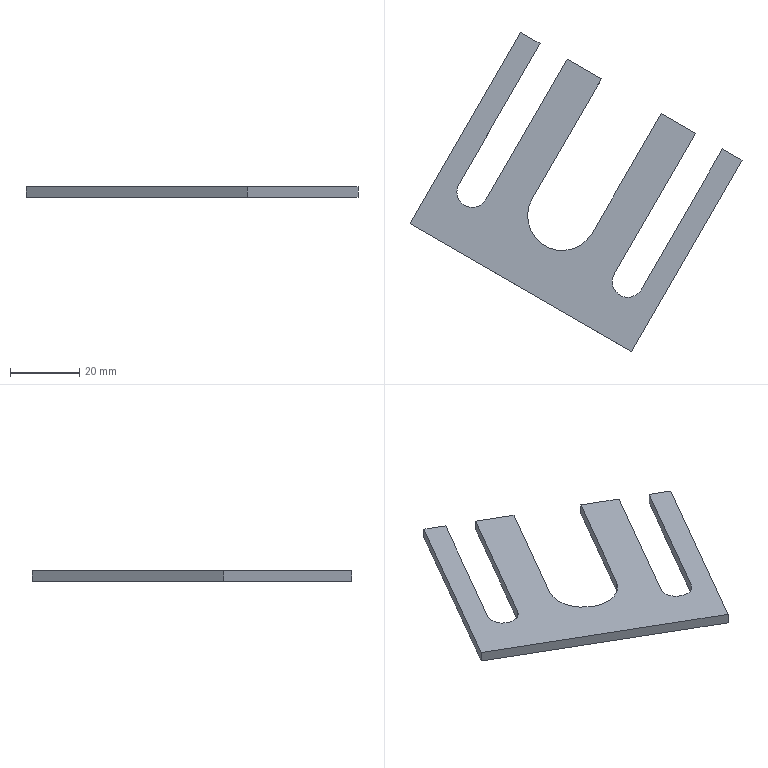Component | SolidWorks | KLHFH018AdjustmentShim-1 | 1 solid | 18 faces | box 96.09 x 92.43 x 3 mm | volume 8608 mm3 | plane 15 | cylinder 3 | commonest cylinder face diameters 9 x2 20 x1 | material AISI 304
build123d program:
from build123d import *

# Parameters (mm, degrees)
SKETCH1_W           = 74
SKETCH1_H           = 64
BOSS_EXTRUDE1_DEPTH = 1.5
SKETCH2_R           = 8
CUT_EXTRUDE1_DEPTH  = 50.01
M8_TAPPED_HOLE1_D   = 6.8
CIRPATTERN1_COUNT   = 6
CUT_EXTRUDE2_DEPTH  = 50.01


with BuildPart() as part:
    # Sketch1 → Boss-Extrude1 (new, symmetric)
    with BuildSketch(Plane.XY):
        Rectangle(SKETCH1_W, SKETCH1_H)
    extrude(amount=BOSS_EXTRUDE1_DEPTH, both=True)

    # Sketch2 → Cut-Extrude1 (cut, through all)
    with BuildSketch(Plane.XY.offset(1.5)):
        Circle(SKETCH2_R)
    extrude(amount=-CUT_EXTRUDE1_DEPTH, mode=Mode.SUBTRACT)

    # M8 Tapped Hole1 (through all)
    with Locations(Plane(origin=(0, 0, -1.5), x_dir=(-1, 0, 0), z_dir=(0, 0, -1))):
        with Locations((-25.981, 15)):
            m8_tapped_hole1 = Hole(M8_TAPPED_HOLE1_D / 2)

    # CirPattern1: M8 Tapped Hole1 ×6 about axis, 2 skipped
    cirpattern1_axis = Axis((0, 0, -1.5), (0, 0, 1))
    add([m8_tapped_hole1.rotate(cirpattern1_axis, i * 360 / CIRPATTERN1_COUNT) for i in range(1, CIRPATTERN1_COUNT) if i not in (1, 4)], mode=Mode.SUBTRACT)

    # Sketch7 → Cut-Extrude2 (cut, through all)
    with BuildSketch(Plane.XY.offset(1.5)):
        with BuildLine():
            Line((-21.481, 15), (-21.481, -32))
            ThreePointArc((-21.481, -32), (-25.981, -36.5), (-30.481, -32))
            Line((-30.481, -32), (-30.481, 15))
            ThreePointArc((-30.481, 15), (-25.981, 19.5), (-21.481, 15))
        make_face()
        with BuildLine():
            Line((30.481, 15), (30.481, -32))
            ThreePointArc((30.481, -32), (25.981, -36.5), (21.481, -32))
            Line((21.481, -32), (21.481, 15))
            ThreePointArc((21.481, 15), (25.981, 19.5), (30.481, 15))
        make_face()
        with BuildLine():
            Line((10, 8), (10, -32))
            ThreePointArc((10, -32), (0, -42), (-10, -32))
            Line((-10, -32), (-10, 8))
            ThreePointArc((-10, 8), (0, 18), (10, 8))
        make_face()
    extrude(amount=-CUT_EXTRUDE2_DEPTH, mode=Mode.SUBTRACT)


solid = part.part

# Placed as in the assembly
solid = solid.moved(Location((90.792, 157.737, -442.5), (-180, 0, 30)))
STEP:
#1=CARTESIAN_POINT('',(3.863,7.498,-17.362));
#2=VERTEX_POINT('',#1);
#3=CARTESIAN_POINT('',(3.472,7.724,-17.362));
#4=VERTEX_POINT('',#3);
#5=CARTESIAN_POINT('',(2.943,8.03,-17.362));
#6=DIRECTION('',(-0.866,0.5,0.));
#7=VECTOR('',#6,39.37);
#8=LINE('',#5,#7);
#9=EDGE_CURVE('',#2,#4,#8,.T.);
#10=ORIENTED_EDGE('',*,*,#9,.F.);
#11=CARTESIAN_POINT('',(3.863,7.498,-17.48));
#12=VERTEX_POINT('',#11);
#13=CARTESIAN_POINT('',(3.863,7.498,-17.48));
#14=DIRECTION('',(0.,0.,1.));
#15=VECTOR('',#14,39.37);
#16=LINE('',#13,#15);
#17=EDGE_CURVE('',#12,#2,#16,.T.);
#18=ORIENTED_EDGE('',*,*,#17,.F.);
#19=CARTESIAN_POINT('',(3.472,7.724,-17.48));
#20=VERTEX_POINT('',#19);
#21=CARTESIAN_POINT('',(2.943,8.03,-17.48));
#22=DIRECTION('',(-0.866,0.5,0.));
#23=VECTOR('',#22,39.37);
#24=LINE('',#21,#23);
#25=EDGE_CURVE('',#12,#20,#24,.T.);
#26=ORIENTED_EDGE('',*,*,#25,.T.);
#27=CARTESIAN_POINT('',(3.472,7.724,-17.48));
#28=DIRECTION('',(0.,0.,1.));
#29=VECTOR('',#28,39.37);
#30=LINE('',#27,#29);
#31=EDGE_CURVE('',#20,#4,#30,.T.);
#32=ORIENTED_EDGE('',*,*,#31,.T.);
#33=EDGE_LOOP('',(#10,#18,#26,#32));
#34=FACE_OUTER_BOUND('',#33,.T.);
#35=CARTESIAN_POINT('',(2.943,8.03,-17.362));
#36=DIRECTION('',(-0.5,-0.866,0.));
#37=DIRECTION('',(0.866,-0.5,0.));
#38=AXIS2_PLACEMENT_3D('',#35,#36,#37);
#39=PLANE('',#38);
#40=ADVANCED_FACE('',(#34),#39,.F.);
#41=CARTESIAN_POINT('',(3.165,7.901,-17.362));
#42=VERTEX_POINT('',#41);
#43=CARTESIAN_POINT('',(2.943,8.03,-17.362));
#44=VERTEX_POINT('',#43);
#45=CARTESIAN_POINT('',(2.943,8.03,-17.362));
#46=DIRECTION('',(-0.866,0.5,0.));
#47=VECTOR('',#46,39.37);
#48=LINE('',#45,#47);
#49=EDGE_CURVE('',#42,#44,#48,.T.);
#50=ORIENTED_EDGE('',*,*,#49,.F.);
#51=CARTESIAN_POINT('',(3.165,7.901,-17.48));
#52=VERTEX_POINT('',#51);
#53=CARTESIAN_POINT('',(3.165,7.901,-17.48));
#54=DIRECTION('',(0.,0.,1.));
#55=VECTOR('',#54,39.37);
#56=LINE('',#53,#55);
#57=EDGE_CURVE('',#52,#42,#56,.T.);
#58=ORIENTED_EDGE('',*,*,#57,.F.);
#59=CARTESIAN_POINT('',(2.943,8.03,-17.48));
#60=VERTEX_POINT('',#59);
#61=CARTESIAN_POINT('',(2.943,8.03,-17.48));
#62=DIRECTION('',(-0.866,0.5,0.));
#63=VECTOR('',#62,39.37);
#64=LINE('',#61,#63);
#65=EDGE_CURVE('',#52,#60,#64,.T.);
#66=ORIENTED_EDGE('',*,*,#65,.T.);
#67=CARTESIAN_POINT('',(2.943,8.03,-17.362));
#68=DIRECTION('',(0.,0.,-1.));
#69=VECTOR('',#68,39.37);
#70=LINE('',#67,#69);
#71=EDGE_CURVE('',#44,#60,#70,.T.);
#72=ORIENTED_EDGE('',*,*,#71,.F.);
#73=EDGE_LOOP('',(#50,#58,#66,#72));
#74=FACE_OUTER_BOUND('',#73,.T.);
#75=CARTESIAN_POINT('',(2.943,8.03,-17.362));
#76=DIRECTION('',(-0.5,-0.866,0.));
#77=DIRECTION('',(0.866,-0.5,0.));
#78=AXIS2_PLACEMENT_3D('',#75,#76,#77);
#79=PLANE('',#78);
#80=ADVANCED_FACE('',(#74),#79,.F.);
#81=CARTESIAN_POINT('',(4.937,6.878,-17.48));
#82=VERTEX_POINT('',#81);
#83=CARTESIAN_POINT('',(4.545,7.104,-17.48));
#84=VERTEX_POINT('',#83);
#85=CARTESIAN_POINT('',(2.943,8.03,-17.48));
#86=DIRECTION('',(-0.866,0.5,0.));
#87=VECTOR('',#86,39.37);
#88=LINE('',#85,#87);
#89=EDGE_CURVE('',#82,#84,#88,.T.);
#90=ORIENTED_EDGE('',*,*,#89,.T.);
#91=CARTESIAN_POINT('',(4.545,7.104,-17.362));
#92=VERTEX_POINT('',#91);
#93=CARTESIAN_POINT('',(4.545,7.104,-17.48));
#94=DIRECTION('',(0.,0.,1.));
#95=VECTOR('',#94,39.37);
#96=LINE('',#93,#95);
#97=EDGE_CURVE('',#84,#92,#96,.T.);
#98=ORIENTED_EDGE('',*,*,#97,.T.);
#99=CARTESIAN_POINT('',(4.937,6.878,-17.362));
#100=VERTEX_POINT('',#99);
#101=CARTESIAN_POINT('',(2.943,8.03,-17.362));
#102=DIRECTION('',(-0.866,0.5,0.));
#103=VECTOR('',#102,39.37);
#104=LINE('',#101,#103);
#105=EDGE_CURVE('',#100,#92,#104,.T.);
#106=ORIENTED_EDGE('',*,*,#105,.F.);
#107=CARTESIAN_POINT('',(4.937,6.878,-17.48));
#108=DIRECTION('',(0.,0.,1.));
#109=VECTOR('',#108,39.37);
#110=LINE('',#107,#109);
#111=EDGE_CURVE('',#82,#100,#110,.T.);
#112=ORIENTED_EDGE('',*,*,#111,.F.);
#113=EDGE_LOOP('',(#90,#98,#106,#112));
#114=FACE_OUTER_BOUND('',#113,.T.);
#115=CARTESIAN_POINT('',(2.943,8.03,-17.362));
#116=DIRECTION('',(-0.5,-0.866,0.));
#117=DIRECTION('',(0.866,-0.5,0.));
#118=AXIS2_PLACEMENT_3D('',#115,#116,#117);
#119=PLANE('',#118);
#120=ADVANCED_FACE('',(#114),#119,.F.);
#121=CARTESIAN_POINT('',(4.206,4.391,-17.48));
#122=VERTEX_POINT('',#121);
#123=CARTESIAN_POINT('',(5.466,6.573,-17.48));
#124=VERTEX_POINT('',#123);
#125=CARTESIAN_POINT('',(4.206,4.391,-17.48));
#126=DIRECTION('',(0.5,0.866,0.));
#127=VECTOR('',#126,39.37);
#128=LINE('',#125,#127);
#129=EDGE_CURVE('',#122,#124,#128,.T.);
#130=ORIENTED_EDGE('',*,*,#129,.T.);
#131=CARTESIAN_POINT('',(5.466,6.573,-17.362));
#132=VERTEX_POINT('',#131);
#133=CARTESIAN_POINT('',(5.466,6.573,-17.362));
#134=DIRECTION('',(0.,0.,-1.));
#135=VECTOR('',#134,39.37);
#136=LINE('',#133,#135);
#137=EDGE_CURVE('',#132,#124,#136,.T.);
#138=ORIENTED_EDGE('',*,*,#137,.F.);
#139=CARTESIAN_POINT('',(4.206,4.391,-17.362));
#140=VERTEX_POINT('',#139);
#141=CARTESIAN_POINT('',(4.206,4.391,-17.362));
#142=DIRECTION('',(0.5,0.866,0.));
#143=VECTOR('',#142,39.37);
#144=LINE('',#141,#143);
#145=EDGE_CURVE('',#140,#132,#144,.T.);
#146=ORIENTED_EDGE('',*,*,#145,.F.);
#147=CARTESIAN_POINT('',(4.206,4.391,-17.362));
#148=DIRECTION('',(0.,0.,-1.));
#149=VECTOR('',#148,39.37);
#150=LINE('',#147,#149);
#151=EDGE_CURVE('',#140,#122,#150,.T.);
#152=ORIENTED_EDGE('',*,*,#151,.T.);
#153=EDGE_LOOP('',(#130,#138,#146,#152));
#154=FACE_OUTER_BOUND('',#153,.T.);
#155=CARTESIAN_POINT('',(4.206,4.391,-17.362));
#156=DIRECTION('',(-0.866,0.5,0.));
#157=DIRECTION('',(-0.5,-0.866,0.));
#158=AXIS2_PLACEMENT_3D('',#155,#156,#157);
#159=PLANE('',#158);
#160=ADVANCED_FACE('',(#154),#159,.F.);
#161=CARTESIAN_POINT('',(5.244,6.701,-17.48));
#162=VERTEX_POINT('',#161);
#163=CARTESIAN_POINT('',(2.943,8.03,-17.48));
#164=DIRECTION('',(-0.866,0.5,0.));
#165=VECTOR('',#164,39.37);
#166=LINE('',#163,#165);
#167=EDGE_CURVE('',#124,#162,#166,.T.);
#168=ORIENTED_EDGE('',*,*,#167,.T.);
#169=CARTESIAN_POINT('',(5.244,6.701,-17.362));
#170=VERTEX_POINT('',#169);
#171=CARTESIAN_POINT('',(5.244,6.701,-17.48));
#172=DIRECTION('',(0.,0.,1.));
#173=VECTOR('',#172,39.37);
#174=LINE('',#171,#173);
#175=EDGE_CURVE('',#162,#170,#174,.T.);
#176=ORIENTED_EDGE('',*,*,#175,.T.);
#177=CARTESIAN_POINT('',(2.943,8.03,-17.362));
#178=DIRECTION('',(-0.866,0.5,0.));
#179=VECTOR('',#178,39.37);
#180=LINE('',#177,#179);
#181=EDGE_CURVE('',#132,#170,#180,.T.);
#182=ORIENTED_EDGE('',*,*,#181,.F.);
#183=ORIENTED_EDGE('',*,*,#137,.T.);
#184=EDGE_LOOP('',(#168,#176,#182,#183));
#185=FACE_OUTER_BOUND('',#184,.T.);
#186=CARTESIAN_POINT('',(2.943,8.03,-17.362));
#187=DIRECTION('',(-0.5,-0.866,0.));
#188=DIRECTION('',(0.866,-0.5,0.));
#189=AXIS2_PLACEMENT_3D('',#186,#187,#188);
#190=PLANE('',#189);
#191=ADVANCED_FACE('',(#185),#190,.F.);
#192=CARTESIAN_POINT('',(1.683,5.847,-17.48));
#193=VERTEX_POINT('',#192);
#194=CARTESIAN_POINT('',(1.683,5.847,-17.48));
#195=DIRECTION('',(-0.5,-0.866,0.));
#196=VECTOR('',#195,39.37);
#197=LINE('',#194,#196);
#198=EDGE_CURVE('',#60,#193,#197,.T.);
#199=ORIENTED_EDGE('',*,*,#198,.T.);
#200=CARTESIAN_POINT('',(1.683,5.847,-17.362));
#201=VERTEX_POINT('',#200);
#202=CARTESIAN_POINT('',(1.683,5.847,-17.362));
#203=DIRECTION('',(0.,0.,-1.));
#204=VECTOR('',#203,39.37);
#205=LINE('',#202,#204);
#206=EDGE_CURVE('',#201,#193,#205,.T.);
#207=ORIENTED_EDGE('',*,*,#206,.F.);
#208=CARTESIAN_POINT('',(1.683,5.847,-17.362));
#209=DIRECTION('',(-0.5,-0.866,0.));
#210=VECTOR('',#209,39.37);
#211=LINE('',#208,#210);
#212=EDGE_CURVE('',#44,#201,#211,.T.);
#213=ORIENTED_EDGE('',*,*,#212,.F.);
#214=ORIENTED_EDGE('',*,*,#71,.T.);
#215=EDGE_LOOP('',(#199,#207,#213,#214));
#216=FACE_OUTER_BOUND('',#215,.T.);
#217=CARTESIAN_POINT('',(1.683,5.847,-17.362));
#218=DIRECTION('',(0.866,-0.5,0.));
#219=DIRECTION('',(0.5,0.866,0.));
#220=AXIS2_PLACEMENT_3D('',#217,#218,#219);
#221=PLANE('',#220);
#222=ADVANCED_FACE('',(#216),#221,.F.);
#223=CARTESIAN_POINT('',(1.683,5.847,-17.48));
#224=DIRECTION('',(0.866,-0.5,0.));
#225=VECTOR('',#224,39.37);
#226=LINE('',#223,#225);
#227=EDGE_CURVE('',#193,#122,#226,.T.);
#228=ORIENTED_EDGE('',*,*,#227,.T.);
#229=ORIENTED_EDGE('',*,*,#151,.F.);
#230=CARTESIAN_POINT('',(1.683,5.847,-17.362));
#231=DIRECTION('',(0.866,-0.5,0.));
#232=VECTOR('',#231,39.37);
#233=LINE('',#230,#232);
#234=EDGE_CURVE('',#201,#140,#233,.T.);
#235=ORIENTED_EDGE('',*,*,#234,.F.);
#236=ORIENTED_EDGE('',*,*,#206,.T.);
#237=EDGE_LOOP('',(#228,#229,#235,#236));
#238=FACE_OUTER_BOUND('',#237,.T.);
#239=CARTESIAN_POINT('',(1.683,5.847,-17.362));
#240=DIRECTION('',(0.5,0.866,0.));
#241=DIRECTION('',(-0.866,0.5,0.));
#242=AXIS2_PLACEMENT_3D('',#239,#240,#241);
#243=PLANE('',#242);
#244=ADVANCED_FACE('',(#238),#243,.F.);
#245=CARTESIAN_POINT('',(3.076,6.134,-17.362));
#246=VERTEX_POINT('',#245);
#247=CARTESIAN_POINT('',(3.758,5.74,-17.362));
#248=VERTEX_POINT('',#247);
#249=CARTESIAN_POINT('',(3.417,5.937,-17.362));
#250=DIRECTION('',(0.,0.,1.));
#251=DIRECTION('',(-0.866,0.5,0.));
#252=AXIS2_PLACEMENT_3D('',#249,#250,#251);
#253=CIRCLE('',#252,0.3937);
#254=EDGE_CURVE('',#246,#248,#253,.T.);
#255=ORIENTED_EDGE('',*,*,#254,.F.);
#256=CARTESIAN_POINT('',(3.076,6.134,-17.362));
#257=DIRECTION('',(-0.5,-0.866,0.));
#258=VECTOR('',#257,39.37);
#259=LINE('',#256,#258);
#260=EDGE_CURVE('',#2,#246,#259,.T.);
#261=ORIENTED_EDGE('',*,*,#260,.F.);
#262=ORIENTED_EDGE('',*,*,#9,.T.);
#263=CARTESIAN_POINT('',(2.547,6.122,-17.362));
#264=VERTEX_POINT('',#263);
#265=CARTESIAN_POINT('',(2.547,6.122,-17.362));
#266=DIRECTION('',(0.5,0.866,0.));
#267=VECTOR('',#266,39.37);
#268=LINE('',#265,#267);
#269=EDGE_CURVE('',#264,#4,#268,.T.);
#270=ORIENTED_EDGE('',*,*,#269,.F.);
#271=CARTESIAN_POINT('',(2.24,6.299,-17.362));
#272=VERTEX_POINT('',#271);
#273=CARTESIAN_POINT('',(2.393,6.21,-17.362));
#274=DIRECTION('',(0.,0.,1.));
#275=DIRECTION('',(-0.866,0.5,0.));
#276=AXIS2_PLACEMENT_3D('',#273,#274,#275);
#277=CIRCLE('',#276,0.1772);
#278=EDGE_CURVE('',#272,#264,#277,.T.);
#279=ORIENTED_EDGE('',*,*,#278,.F.);
#280=CARTESIAN_POINT('',(2.24,6.299,-17.362));
#281=DIRECTION('',(-0.5,-0.866,0.));
#282=VECTOR('',#281,39.37);
#283=LINE('',#280,#282);
#284=EDGE_CURVE('',#42,#272,#283,.T.);
#285=ORIENTED_EDGE('',*,*,#284,.F.);
#286=ORIENTED_EDGE('',*,*,#49,.T.);
#287=ORIENTED_EDGE('',*,*,#212,.T.);
#288=ORIENTED_EDGE('',*,*,#234,.T.);
#289=ORIENTED_EDGE('',*,*,#145,.T.);
#290=ORIENTED_EDGE('',*,*,#181,.T.);
#291=CARTESIAN_POINT('',(4.318,5.099,-17.362));
#292=VERTEX_POINT('',#291);
#293=CARTESIAN_POINT('',(4.318,5.099,-17.362));
#294=DIRECTION('',(0.5,0.866,0.));
#295=VECTOR('',#294,39.37);
#296=LINE('',#293,#295);
#297=EDGE_CURVE('',#292,#170,#296,.T.);
#298=ORIENTED_EDGE('',*,*,#297,.F.);
#299=CARTESIAN_POINT('',(4.012,5.276,-17.362));
#300=VERTEX_POINT('',#299);
#301=CARTESIAN_POINT('',(4.165,5.187,-17.362));
#302=DIRECTION('',(0.,0.,1.));
#303=DIRECTION('',(-0.866,0.5,0.));
#304=AXIS2_PLACEMENT_3D('',#301,#302,#303);
#305=CIRCLE('',#304,0.1772);
#306=EDGE_CURVE('',#300,#292,#305,.T.);
#307=ORIENTED_EDGE('',*,*,#306,.F.);
#308=CARTESIAN_POINT('',(4.012,5.276,-17.362));
#309=DIRECTION('',(-0.5,-0.866,0.));
#310=VECTOR('',#309,39.37);
#311=LINE('',#308,#310);
#312=EDGE_CURVE('',#100,#300,#311,.T.);
#313=ORIENTED_EDGE('',*,*,#312,.F.);
#314=ORIENTED_EDGE('',*,*,#105,.T.);
#315=CARTESIAN_POINT('',(3.758,5.74,-17.362));
#316=DIRECTION('',(0.5,0.866,0.));
#317=VECTOR('',#316,39.37);
#318=LINE('',#315,#317);
#319=EDGE_CURVE('',#248,#92,#318,.T.);
#320=ORIENTED_EDGE('',*,*,#319,.F.);
#321=EDGE_LOOP('',(#255,#261,#262,#270,#279,#285,#286,#287,#288,#289,#290,#298,#307,#313,#314,#320));
#322=FACE_OUTER_BOUND('',#321,.T.);
#323=CARTESIAN_POINT('',(3.574,6.21,-17.362));
#324=DIRECTION('',(0.,0.,-1.));
#325=DIRECTION('',(0.866,-0.5,0.));
#326=AXIS2_PLACEMENT_3D('',#323,#324,#325);
#327=PLANE('',#326);
#328=ADVANCED_FACE('',(#322),#327,.F.);
#329=CARTESIAN_POINT('',(3.076,6.134,-17.48));
#330=VERTEX_POINT('',#329);
#331=CARTESIAN_POINT('',(3.076,6.134,-17.48));
#332=DIRECTION('',(-0.5,-0.866,0.));
#333=VECTOR('',#332,39.37);
#334=LINE('',#331,#333);
#335=EDGE_CURVE('',#12,#330,#334,.T.);
#336=ORIENTED_EDGE('',*,*,#335,.T.);
#337=CARTESIAN_POINT('',(3.758,5.74,-17.48));
#338=VERTEX_POINT('',#337);
#339=CARTESIAN_POINT('',(3.417,5.937,-17.48));
#340=DIRECTION('',(0.,0.,1.));
#341=DIRECTION('',(-0.866,0.5,0.));
#342=AXIS2_PLACEMENT_3D('',#339,#340,#341);
#343=CIRCLE('',#342,0.3937);
#344=EDGE_CURVE('',#330,#338,#343,.T.);
#345=ORIENTED_EDGE('',*,*,#344,.T.);
#346=CARTESIAN_POINT('',(3.758,5.74,-17.48));
#347=DIRECTION('',(0.5,0.866,0.));
#348=VECTOR('',#347,39.37);
#349=LINE('',#346,#348);
#350=EDGE_CURVE('',#338,#84,#349,.T.);
#351=ORIENTED_EDGE('',*,*,#350,.T.);
#352=ORIENTED_EDGE('',*,*,#89,.F.);
#353=CARTESIAN_POINT('',(4.012,5.276,-17.48));
#354=VERTEX_POINT('',#353);
#355=CARTESIAN_POINT('',(4.012,5.276,-17.48));
#356=DIRECTION('',(-0.5,-0.866,0.));
#357=VECTOR('',#356,39.37);
#358=LINE('',#355,#357);
#359=EDGE_CURVE('',#82,#354,#358,.T.);
#360=ORIENTED_EDGE('',*,*,#359,.T.);
#361=CARTESIAN_POINT('',(4.318,5.099,-17.48));
#362=VERTEX_POINT('',#361);
#363=CARTESIAN_POINT('',(4.165,5.187,-17.48));
#364=DIRECTION('',(0.,0.,1.));
#365=DIRECTION('',(-0.866,0.5,0.));
#366=AXIS2_PLACEMENT_3D('',#363,#364,#365);
#367=CIRCLE('',#366,0.1772);
#368=EDGE_CURVE('',#354,#362,#367,.T.);
#369=ORIENTED_EDGE('',*,*,#368,.T.);
#370=CARTESIAN_POINT('',(4.318,5.099,-17.48));
#371=DIRECTION('',(0.5,0.866,0.));
#372=VECTOR('',#371,39.37);
#373=LINE('',#370,#372);
#374=EDGE_CURVE('',#362,#162,#373,.T.);
#375=ORIENTED_EDGE('',*,*,#374,.T.);
#376=ORIENTED_EDGE('',*,*,#167,.F.);
#377=ORIENTED_EDGE('',*,*,#129,.F.);
#378=ORIENTED_EDGE('',*,*,#227,.F.);
#379=ORIENTED_EDGE('',*,*,#198,.F.);
#380=ORIENTED_EDGE('',*,*,#65,.F.);
#381=CARTESIAN_POINT('',(2.24,6.299,-17.48));
#382=VERTEX_POINT('',#381);
#383=CARTESIAN_POINT('',(2.24,6.299,-17.48));
#384=DIRECTION('',(-0.5,-0.866,0.));
#385=VECTOR('',#384,39.37);
#386=LINE('',#383,#385);
#387=EDGE_CURVE('',#52,#382,#386,.T.);
#388=ORIENTED_EDGE('',*,*,#387,.T.);
#389=CARTESIAN_POINT('',(2.547,6.122,-17.48));
#390=VERTEX_POINT('',#389);
#391=CARTESIAN_POINT('',(2.393,6.21,-17.48));
#392=DIRECTION('',(0.,0.,1.));
#393=DIRECTION('',(-0.866,0.5,0.));
#394=AXIS2_PLACEMENT_3D('',#391,#392,#393);
#395=CIRCLE('',#394,0.1772);
#396=EDGE_CURVE('',#382,#390,#395,.T.);
#397=ORIENTED_EDGE('',*,*,#396,.T.);
#398=CARTESIAN_POINT('',(2.547,6.122,-17.48));
#399=DIRECTION('',(0.5,0.866,0.));
#400=VECTOR('',#399,39.37);
#401=LINE('',#398,#400);
#402=EDGE_CURVE('',#390,#20,#401,.T.);
#403=ORIENTED_EDGE('',*,*,#402,.T.);
#404=ORIENTED_EDGE('',*,*,#25,.F.);
#405=EDGE_LOOP('',(#336,#345,#351,#352,#360,#369,#375,#376,#377,#378,#379,#380,#388,#397,#403,#404));
#406=FACE_OUTER_BOUND('',#405,.T.);
#407=CARTESIAN_POINT('',(3.574,6.21,-17.48));
#408=DIRECTION('',(0.,0.,-1.));
#409=DIRECTION('',(0.866,-0.5,0.));
#410=AXIS2_PLACEMENT_3D('',#407,#408,#409);
#411=PLANE('',#410);
#412=ADVANCED_FACE('',(#406),#411,.T.);
#413=ORIENTED_EDGE('',*,*,#306,.T.);
#414=CARTESIAN_POINT('',(4.318,5.099,-17.48));
#415=DIRECTION('',(0.,0.,1.));
#416=VECTOR('',#415,39.37);
#417=LINE('',#414,#416);
#418=EDGE_CURVE('',#362,#292,#417,.T.);
#419=ORIENTED_EDGE('',*,*,#418,.F.);
#420=ORIENTED_EDGE('',*,*,#368,.F.);
#421=CARTESIAN_POINT('',(4.012,5.276,-17.48));
#422=DIRECTION('',(0.,0.,1.));
#423=VECTOR('',#422,39.37);
#424=LINE('',#421,#423);
#425=EDGE_CURVE('',#354,#300,#424,.T.);
#426=ORIENTED_EDGE('',*,*,#425,.T.);
#427=EDGE_LOOP('',(#413,#419,#420,#426));
#428=FACE_OUTER_BOUND('',#427,.T.);
#429=CARTESIAN_POINT('',(4.165,5.187,-17.48));
#430=DIRECTION('',(0.,0.,1.));
#431=DIRECTION('',(-0.866,0.5,0.));
#432=AXIS2_PLACEMENT_3D('',#429,#430,#431);
#433=CYLINDRICAL_SURFACE('',#432,0.1772);
#434=ADVANCED_FACE('',(#428),#433,.F.);
#435=ORIENTED_EDGE('',*,*,#312,.T.);
#436=ORIENTED_EDGE('',*,*,#425,.F.);
#437=ORIENTED_EDGE('',*,*,#359,.F.);
#438=ORIENTED_EDGE('',*,*,#111,.T.);
#439=EDGE_LOOP('',(#435,#436,#437,#438));
#440=FACE_OUTER_BOUND('',#439,.T.);
#441=CARTESIAN_POINT('',(4.012,5.276,-17.48));
#442=DIRECTION('',(-0.866,0.5,0.));
#443=DIRECTION('',(-0.5,-0.866,0.));
#444=AXIS2_PLACEMENT_3D('',#441,#442,#443);
#445=PLANE('',#444);
#446=ADVANCED_FACE('',(#440),#445,.F.);
#447=ORIENTED_EDGE('',*,*,#297,.T.);
#448=ORIENTED_EDGE('',*,*,#175,.F.);
#449=ORIENTED_EDGE('',*,*,#374,.F.);
#450=ORIENTED_EDGE('',*,*,#418,.T.);
#451=EDGE_LOOP('',(#447,#448,#449,#450));
#452=FACE_OUTER_BOUND('',#451,.T.);
#453=CARTESIAN_POINT('',(4.318,5.099,-17.48));
#454=DIRECTION('',(0.866,-0.5,0.));
#455=DIRECTION('',(0.5,0.866,0.));
#456=AXIS2_PLACEMENT_3D('',#453,#454,#455);
#457=PLANE('',#456);
#458=ADVANCED_FACE('',(#452),#457,.F.);
#459=ORIENTED_EDGE('',*,*,#278,.T.);
#460=CARTESIAN_POINT('',(2.547,6.122,-17.48));
#461=DIRECTION('',(0.,0.,1.));
#462=VECTOR('',#461,39.37);
#463=LINE('',#460,#462);
#464=EDGE_CURVE('',#390,#264,#463,.T.);
#465=ORIENTED_EDGE('',*,*,#464,.F.);
#466=ORIENTED_EDGE('',*,*,#396,.F.);
#467=CARTESIAN_POINT('',(2.24,6.299,-17.48));
#468=DIRECTION('',(0.,0.,1.));
#469=VECTOR('',#468,39.37);
#470=LINE('',#467,#469);
#471=EDGE_CURVE('',#382,#272,#470,.T.);
#472=ORIENTED_EDGE('',*,*,#471,.T.);
#473=EDGE_LOOP('',(#459,#465,#466,#472));
#474=FACE_OUTER_BOUND('',#473,.T.);
#475=CARTESIAN_POINT('',(2.393,6.21,-17.48));
#476=DIRECTION('',(0.,0.,1.));
#477=DIRECTION('',(-0.866,0.5,0.));
#478=AXIS2_PLACEMENT_3D('',#475,#476,#477);
#479=CYLINDRICAL_SURFACE('',#478,0.1772);
#480=ADVANCED_FACE('',(#474),#479,.F.);
#481=ORIENTED_EDGE('',*,*,#284,.T.);
#482=ORIENTED_EDGE('',*,*,#471,.F.);
#483=ORIENTED_EDGE('',*,*,#387,.F.);
#484=ORIENTED_EDGE('',*,*,#57,.T.);
#485=EDGE_LOOP('',(#481,#482,#483,#484));
#486=FACE_OUTER_BOUND('',#485,.T.);
#487=CARTESIAN_POINT('',(2.24,6.299,-17.48));
#488=DIRECTION('',(-0.866,0.5,0.));
#489=DIRECTION('',(-0.5,-0.866,0.));
#490=AXIS2_PLACEMENT_3D('',#487,#488,#489);
#491=PLANE('',#490);
#492=ADVANCED_FACE('',(#486),#491,.F.);
#493=ORIENTED_EDGE('',*,*,#269,.T.);
#494=ORIENTED_EDGE('',*,*,#31,.F.);
#495=ORIENTED_EDGE('',*,*,#402,.F.);
#496=ORIENTED_EDGE('',*,*,#464,.T.);
#497=EDGE_LOOP('',(#493,#494,#495,#496));
#498=FACE_OUTER_BOUND('',#497,.T.);
#499=CARTESIAN_POINT('',(2.547,6.122,-17.48));
#500=DIRECTION('',(0.866,-0.5,0.));
#501=DIRECTION('',(0.,0.,1.));
#502=AXIS2_PLACEMENT_3D('',#499,#500,#501);
#503=PLANE('',#502);
#504=ADVANCED_FACE('',(#498),#503,.F.);
#505=ORIENTED_EDGE('',*,*,#254,.T.);
#506=CARTESIAN_POINT('',(3.758,5.74,-17.48));
#507=DIRECTION('',(0.,0.,1.));
#508=VECTOR('',#507,39.37);
#509=LINE('',#506,#508);
#510=EDGE_CURVE('',#338,#248,#509,.T.);
#511=ORIENTED_EDGE('',*,*,#510,.F.);
#512=ORIENTED_EDGE('',*,*,#344,.F.);
#513=CARTESIAN_POINT('',(3.076,6.134,-17.48));
#514=DIRECTION('',(0.,0.,1.));
#515=VECTOR('',#514,39.37);
#516=LINE('',#513,#515);
#517=EDGE_CURVE('',#330,#246,#516,.T.);
#518=ORIENTED_EDGE('',*,*,#517,.T.);
#519=EDGE_LOOP('',(#505,#511,#512,#518));
#520=FACE_OUTER_BOUND('',#519,.T.);
#521=CARTESIAN_POINT('',(3.417,5.937,-17.48));
#522=DIRECTION('',(0.,0.,1.));
#523=DIRECTION('',(-0.866,0.5,0.));
#524=AXIS2_PLACEMENT_3D('',#521,#522,#523);
#525=CYLINDRICAL_SURFACE('',#524,0.3937);
#526=ADVANCED_FACE('',(#520),#525,.F.);
#527=ORIENTED_EDGE('',*,*,#260,.T.);
#528=ORIENTED_EDGE('',*,*,#517,.F.);
#529=ORIENTED_EDGE('',*,*,#335,.F.);
#530=ORIENTED_EDGE('',*,*,#17,.T.);
#531=EDGE_LOOP('',(#527,#528,#529,#530));
#532=FACE_OUTER_BOUND('',#531,.T.);
#533=CARTESIAN_POINT('',(3.076,6.134,-17.48));
#534=DIRECTION('',(-0.866,0.5,0.));
#535=DIRECTION('',(-0.5,-0.866,0.));
#536=AXIS2_PLACEMENT_3D('',#533,#534,#535);
#537=PLANE('',#536);
#538=ADVANCED_FACE('',(#532),#537,.F.);
#539=ORIENTED_EDGE('',*,*,#319,.T.);
#540=ORIENTED_EDGE('',*,*,#97,.F.);
#541=ORIENTED_EDGE('',*,*,#350,.F.);
#542=ORIENTED_EDGE('',*,*,#510,.T.);
#543=EDGE_LOOP('',(#539,#540,#541,#542));
#544=FACE_OUTER_BOUND('',#543,.T.);
#545=CARTESIAN_POINT('',(3.758,5.74,-17.48));
#546=DIRECTION('',(0.866,-0.5,0.));
#547=DIRECTION('',(0.5,0.866,0.));
#548=AXIS2_PLACEMENT_3D('',#545,#546,#547);
#549=PLANE('',#548);
#550=ADVANCED_FACE('',(#544),#549,.F.);
#551=CLOSED_SHELL('',(#40,#80,#120,#160,#191,#222,#244,#328,#412,#434,#446,#458,#480,#492,#504,#526,#538,#550));
#552=MANIFOLD_SOLID_BREP('',#551);
#553=CARTESIAN_POINT('',(0.,0.,0.));
#554=DIRECTION('',(0.,0.,1.));
#555=DIRECTION('',(1.,0.,0.));
#556=AXIS2_PLACEMENT_3D('',#553,#554,#555);
#557=(LENGTH_UNIT()NAMED_UNIT(*)SI_UNIT($,.METRE.));
#558=LENGTH_MEASURE_WITH_UNIT(LENGTH_MEASURE(0.0254),#557);
#559=DIMENSIONAL_EXPONENTS(1.,0.,0.,0.,0.,0.,0.);
#560=(CONVERSION_BASED_UNIT('',#558)LENGTH_UNIT()NAMED_UNIT(#559));
#561=UNCERTAINTY_MEASURE_WITH_UNIT(LENGTH_MEASURE(0.00001),#560,'','');
#562=(NAMED_UNIT(*)PLANE_ANGLE_UNIT()SI_UNIT($,.RADIAN.));
#563=(NAMED_UNIT(*)SI_UNIT($,.STERADIAN.)SOLID_ANGLE_UNIT());
#564=(GEOMETRIC_REPRESENTATION_CONTEXT(3)GLOBAL_UNCERTAINTY_ASSIGNED_CONTEXT((#561))GLOBAL_UNIT_ASSIGNED_CONTEXT((#560,#562,#563))REPRESENTATION_CONTEXT('',''));
#565=ADVANCED_BREP_SHAPE_REPRESENTATION('',(#552,#556),#564);
#566=COLOUR_RGB('',0.7922,0.8196,0.9333);
#567=FILL_AREA_STYLE_COLOUR('',#566);
#568=FILL_AREA_STYLE('',(#567));
#569=SURFACE_STYLE_FILL_AREA(#568);
#570=SURFACE_SIDE_STYLE('',(#569));
#571=SURFACE_STYLE_USAGE(.BOTH.,#570);
#572=PRESENTATION_STYLE_ASSIGNMENT((#571));
#573=STYLED_ITEM('',(#572),#552);
#574=PRESENTATION_LAYER_ASSIGNMENT('','',(#573));
#575=(LENGTH_UNIT()NAMED_UNIT(*)SI_UNIT($,.METRE.));
#576=LENGTH_MEASURE_WITH_UNIT(LENGTH_MEASURE(0.0254),#575);
#577=DIMENSIONAL_EXPONENTS(1.,0.,0.,0.,0.,0.,0.);
#578=(CONVERSION_BASED_UNIT('',#576)LENGTH_UNIT()NAMED_UNIT(#577));
#579=UNCERTAINTY_MEASURE_WITH_UNIT(LENGTH_MEASURE(0.00001),#578,'','');
#580=(NAMED_UNIT(*)PLANE_ANGLE_UNIT()SI_UNIT($,.RADIAN.));
#581=(NAMED_UNIT(*)SI_UNIT($,.STERADIAN.)SOLID_ANGLE_UNIT());
#582=(GEOMETRIC_REPRESENTATION_CONTEXT(3)GLOBAL_UNCERTAINTY_ASSIGNED_CONTEXT((#579))GLOBAL_UNIT_ASSIGNED_CONTEXT((#578,#580,#581))REPRESENTATION_CONTEXT('',''));
#583=MECHANICAL_DESIGN_GEOMETRIC_PRESENTATION_REPRESENTATION('',(#573),#582);